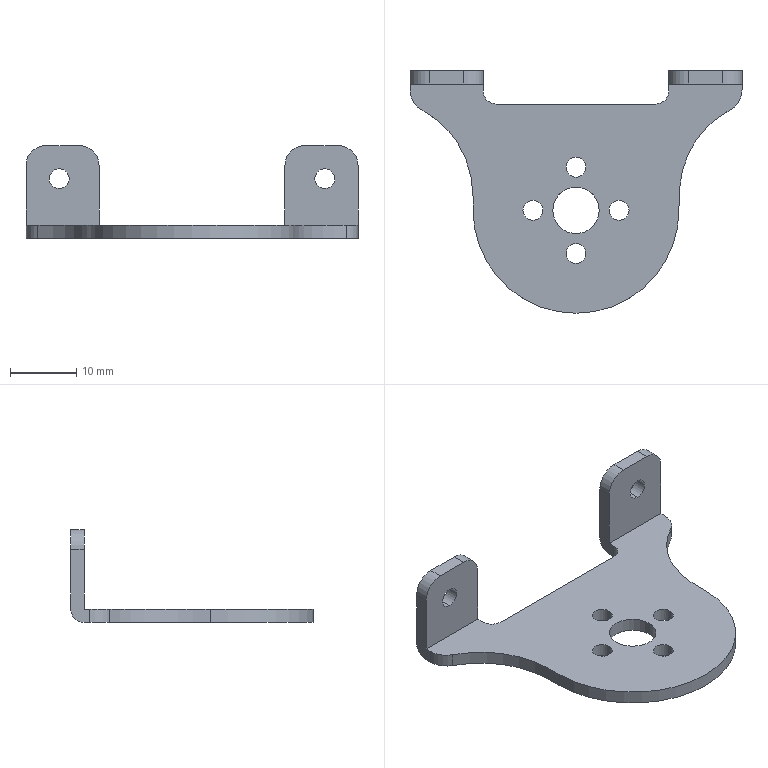Component | SolidWorks | 3-1 | 1 solid | 40 faces | box 50 x 36.5 x 14 mm | volume 2444 mm3 | cylinder 25 | plane 13 | spline 2 | commonest cylinder face diameters 3 x12 7 x4 6 x4 4 x4 31 x1
build123d program:
from build123d import *

# Parameters (mm, degrees)
SKETCH1_R           = 3.5
SKETCH1_R_2         = 1.5
BOSS_EXTRUDE1_DEPTH = 2
SKETCH2_W           = 11
SKETCH2_H           = 2
BOSS_EXTRUDE2_DEPTH = 12
FILLET1_R           = 3
FILLET2_R           = 2
FILLET3_R           = 2
FILLET4_R           = 3.5
SKETCH3_R           = 1.5
CUT_EXTRUDE1_DEPTH  = 21


with BuildPart() as part:
    # Sketch1 → Boss-Extrude1 (new body)
    with BuildSketch(Plane.XY):
        with BuildLine():
            Line((-25, 21), (-14, 21))
            Line((-14, 21), (-14, 16))
            Line((-14, 16), (14, 16))
            Line((14, 16), (14, 21))
            Line((14, 21), (25, 21))
            Line((25, 21), (25, 16))
            add(Edge.make_bspline(
                [(25, 16), (14.96, 11.62), (15.5, 0)],
                knots=[0, 0, 0, 1, 1, 1], degree=2))
            ThreePointArc((15.5, 0), (0, -15.5), (-15.5, 0))
            add(Edge.make_bspline(
                [(-25, 16), (-14.96, 11.62), (-15.5, 0)],
                knots=[0, 0, 0, 1, 1, 1], degree=2))
            Line((-25, 16), (-25, 21))
        make_face()
        Circle(SKETCH1_R, mode=Mode.SUBTRACT)
        with Locations((6.5, 0)):
            Circle(SKETCH1_R_2, mode=Mode.SUBTRACT)
        with Locations((0, -6.5)):
            Circle(SKETCH1_R_2, mode=Mode.SUBTRACT)
        with Locations((-6.5, 0)):
            Circle(SKETCH1_R_2, mode=Mode.SUBTRACT)
        with Locations((0, 6.5)):
            Circle(SKETCH1_R_2, mode=Mode.SUBTRACT)
    extrude(amount=BOSS_EXTRUDE1_DEPTH)

    # Sketch2 → Boss-Extrude2 (add)
    with BuildSketch(Plane.XY.offset(2)):
        with Locations((19.5, 20)):
            Rectangle(SKETCH2_W, SKETCH2_H)
        with Locations((-19.5, 20)):
            Rectangle(SKETCH2_W, SKETCH2_H)
    extrude(amount=BOSS_EXTRUDE2_DEPTH)

    # Fillet1
    fillet1_edges = [part.edges().sort_by_distance(p)[0] for p in [
        (14, 20, 14),
        (25, 20, 14),
        (-25, 20, 14),
        (-14, 20, 14),
    ]]
    fillet(fillet1_edges, radius=FILLET1_R)

    # Fillet2
    fillet2_edges = [part.edges().sort_by_distance(p)[0] for p in [
        (19.5, 21, 0),
        (-19.5, 21, 0),
    ]]
    fillet(fillet2_edges, radius=FILLET2_R)

    # Fillet3
    fillet3_edges = [part.edges().sort_by_distance(p)[0] for p in [
        (-14, 16, 1),
        (14, 16, 1),
    ]]
    fillet(fillet3_edges, radius=FILLET3_R)

    # Fillet4
    fillet4_edges = [part.edges().sort_by_distance(p)[0] for p in [
        (25, 16, 1),
        (-25, 16, 1),
    ]]
    fillet(fillet4_edges, radius=FILLET4_R)

    # Sketch3 → Cut-Extrude1 (cut)
    with BuildSketch(Plane(origin=(0, 21, 0), x_dir=(1, 0, 0), z_dir=(0, 1, 0))):
        with Locations(Location((-20, -9, 0), (0, 0, 270))):
            Circle(SKETCH3_R)
        with Locations(Location((20, -9, 0), (0, 0, 270))):
            Circle(SKETCH3_R)
    extrude(amount=-CUT_EXTRUDE1_DEPTH, mode=Mode.SUBTRACT)


solid = part.part

# Placed as in the assembly
solid = solid.moved(Location((-1.765, -0.369, 24), (0, 0, 0)))